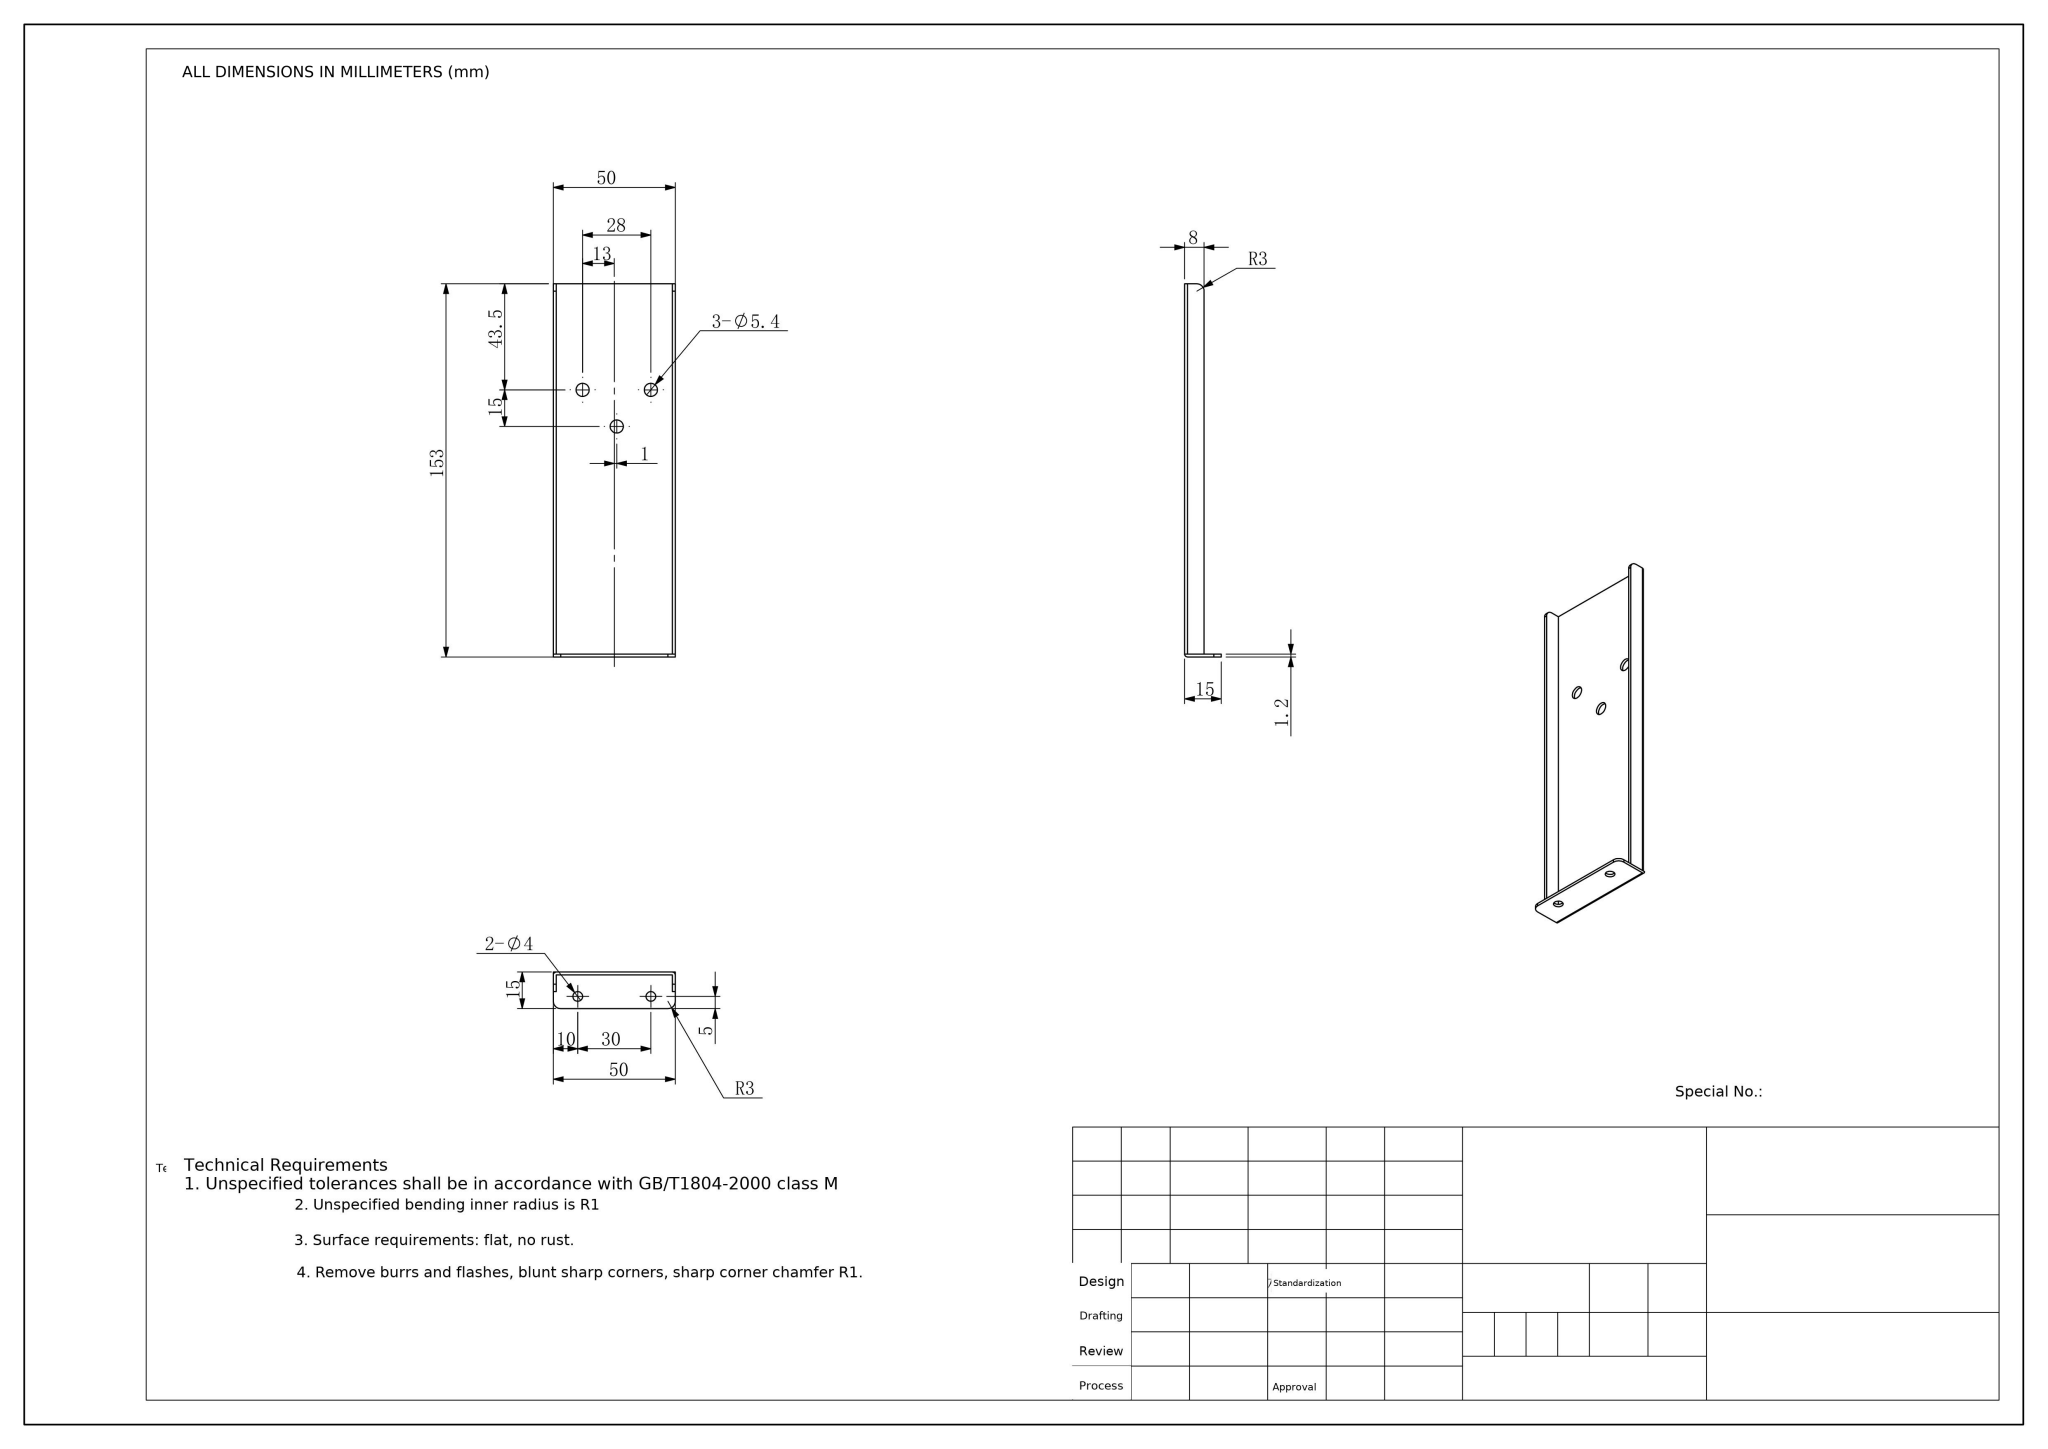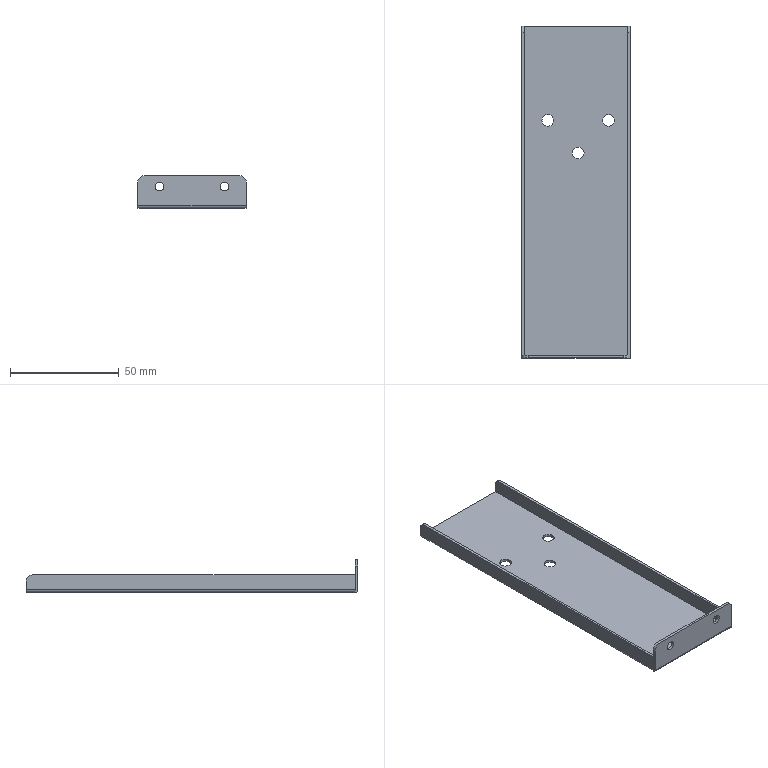Part | NX | mm | 1 solid | 40 faces | box 50 x 153 x 15 mm | volume 12254 mm3 | cylinder 20 | plane 20 | commonest cylinder face diameters 5.4 x6 4 x4 6 x4 2.404 x3 0.004 x3